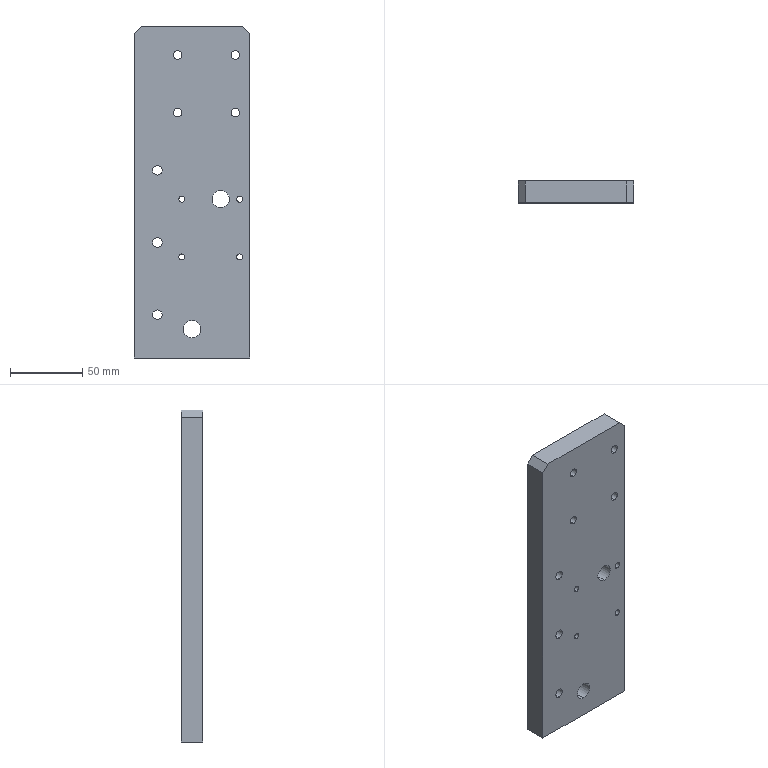Component | SolidWorks | 8TC-A15004-80-05A-1 | 1 solid | 51 faces | box 80 x 15 x 230 mm | volume 266002 mm3 | cylinder 36 | plane 11 | cone 4 | commonest cylinder face diameters 6 x12 4.2 x8 11 x6 6.6 x6 12 x4 | material A3
build123d program:
from build123d import *

# Parameters (mm, degrees)
SKETCH1_W                                       = 80
SKETCH1_H                                       = 230
BOSS_EXTRUDE1_DEPTH                             = 7.5
SKETCH2_R                                       = 6
CUT_EXTRUDE1_DEPTH                              = 244.977
CHAMFER1_SIZE                                   = 5
M6_TAPPED_HOLE1_D                               = 6
M6_TAPPED_HOLE1_DEPTH                           = 17
M6_TAPPED_HOLE1_TIP                             = 1.803
M6_HEX_SOCKET_HEAD_CAP_SCREW_CBORE1_D           = 6.6
M6_HEX_SOCKET_HEAD_CAP_SCREW_CBORE1_CBORE_D     = 11
M6_HEX_SOCKET_HEAD_CAP_SCREW_CBORE1_CBORE_DEPTH = 6.4
M6_TAPPED_HOLE2_D                               = 6
M12_TAPPED_HOLE2_D                              = 12
M5_TAPPED_HOLE1_D                               = 4.2


with BuildPart() as part:
    # Sketch1 → Boss-Extrude1 (new, symmetric)
    with BuildSketch(Plane(origin=(0, 0, 0), x_dir=(1, 0, 0), z_dir=(0, 1, 0))):
        with Locations((40, 115)):
            Rectangle(SKETCH1_W, SKETCH1_H)
    extrude(amount=BOSS_EXTRUDE1_DEPTH, both=True)

    # Sketch2 → Cut-Extrude1 (cut, through all)
    with BuildSketch(Plane(origin=(0, 7.5, 0), x_dir=(1, 0, 0), z_dir=(0, 1, 0))):
        with Locations(Location((60, 110, 0), (0, 0, 270))):
            Circle(SKETCH2_R)
    extrude(amount=-CUT_EXTRUDE1_DEPTH, mode=Mode.SUBTRACT)

    # Chamfer1
    chamfer1_edges = [part.edges().sort_by_distance(p)[0] for p in [
        (0, 0, -230),
        (80, 0, -230),
    ]]
    chamfer(chamfer1_edges, length=CHAMFER1_SIZE)

    # M6 Tapped Hole1
    with Locations(Plane.XY):
        with Locations((20, 0), (60, 0)):
            Hole(M6_TAPPED_HOLE1_D / 2, depth=M6_TAPPED_HOLE1_DEPTH)
            with Locations((0, 0, -(M6_TAPPED_HOLE1_DEPTH + M6_TAPPED_HOLE1_TIP / 2))):  # 118° drill point
                Cone(0, M6_TAPPED_HOLE1_D / 2, M6_TAPPED_HOLE1_TIP, mode=Mode.SUBTRACT)

    # M6 Hex Socket Head Cap Screw CBORE1 (through all)
    with Locations(Plane(origin=(0, -7.5, 0), x_dir=(-1, 0, 0), z_dir=(0, -1, 0))):
        with Locations((-16, 30), (-16, 80), (-16, 130)):
            CounterBoreHole(M6_HEX_SOCKET_HEAD_CAP_SCREW_CBORE1_D / 2, M6_HEX_SOCKET_HEAD_CAP_SCREW_CBORE1_CBORE_D / 2, M6_HEX_SOCKET_HEAD_CAP_SCREW_CBORE1_CBORE_DEPTH)

    # M6 Tapped Hole2 (through all)
    with Locations(Plane(origin=(0, -7.5, 0), x_dir=(-1, 0, 0), z_dir=(0, -1, 0))):
        with Locations((-70, 170), (-30, 210), (-30, 170), (-70, 210)):
            Hole(M6_TAPPED_HOLE2_D / 2)

    # M12 Tapped Hole2 (through all)
    with Locations(Plane(origin=(0, -7.5, 0), x_dir=(-1, 0, 0), z_dir=(0, -1, 0))):
        with Locations((-40, 20)):
            Hole(M12_TAPPED_HOLE2_D / 2)

    # M5 Tapped Hole1 (through all)
    with Locations(Plane(origin=(0, 7.5, 0), x_dir=(1, 0, 0), z_dir=(0, 1, 0))):
        with Locations((73, 70), (73, 110), (33, 110), (33, 70)):
            Hole(M5_TAPPED_HOLE1_D / 2)


solid = part.part

# Placed as in the assembly
solid = solid.moved(Location((0, 0, 40), (180, 0, 0)))